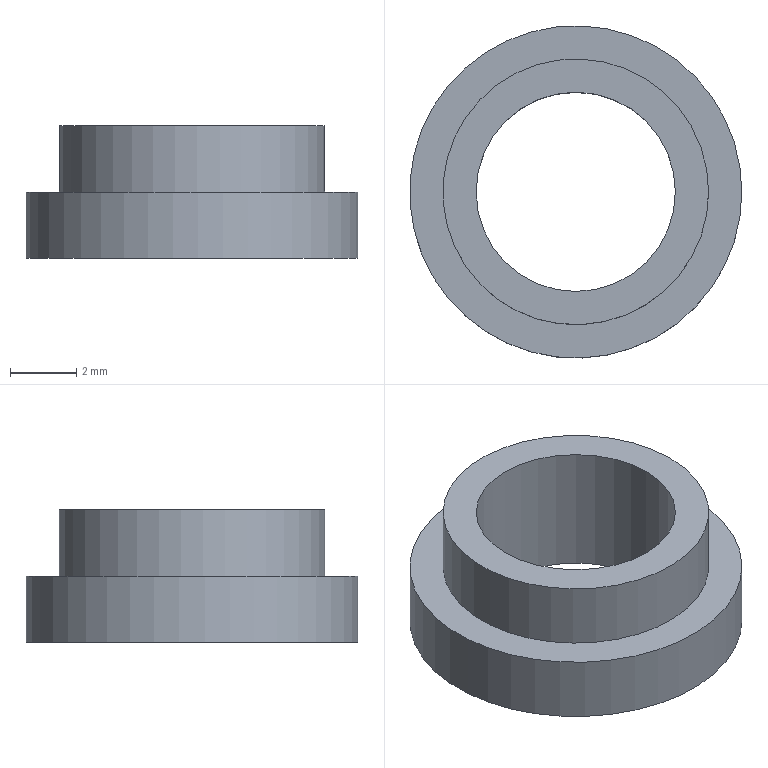Component | NX | BOTTOM_PLATE_CONNECTING_RING | 1 solid | 6 faces | box 10 x 10 x 4 mm | volume 145 mm3 | plane 3 | cylinder 3 | commonest cylinder face diameters 10 x1 8 x1 6 x1
STEP:
#1=CARTESIAN_POINT('',(0.,0.,0.));
#2=DIRECTION('',(0.,0.,1.));
#3=DIRECTION('',(1.,0.,0.));
#4=AXIS2_PLACEMENT_3D('',#1,#2,#3);
#5=CARTESIAN_POINT('',(4.,-10.,123.5));
#6=VERTEX_POINT('',#5);
#7=CARTESIAN_POINT('',(-0.,-10.,123.5));
#8=DIRECTION('',(0.,0.,1.));
#9=DIRECTION('',(1.,0.,0.));
#10=AXIS2_PLACEMENT_3D('',#7,#8,#9);
#11=CIRCLE('',#10,4.);
#12=CARTESIAN_POINT('',(-0.,-10.,123.5));
#13=DIRECTION('',(0.,0.,1.));
#14=DIRECTION('',(1.,0.,0.));
#15=AXIS2_PLACEMENT_3D('',#12,#13,#14);
#16=PLANE('',#15);
#17=CARTESIAN_POINT('',(0.,0.));
#18=DIRECTION('',(1.,0.));
#19=AXIS2_PLACEMENT_2D('',#17,#18);
#20=CIRCLE('',#19,4.);
#21=(GEOMETRIC_REPRESENTATION_CONTEXT(2)PARAMETRIC_REPRESENTATION_CONTEXT()REPRESENTATION_CONTEXT('',''));
#22=DEFINITIONAL_REPRESENTATION('',(#20),#21);
#23=PCURVE('',#16,#22);
#24=CARTESIAN_POINT('',(-0.,-10.,123.5));
#25=DIRECTION('',(0.,0.,1.));
#26=DIRECTION('',(1.,0.,0.));
#27=AXIS2_PLACEMENT_3D('',#24,#25,#26);
#28=CYLINDRICAL_SURFACE('',#27,4.);
#29=CARTESIAN_POINT('',(0.,0.));
#30=DIRECTION('',(1.,0.));
#31=VECTOR('',#30,1.);
#32=LINE('',#29,#31);
#33=(GEOMETRIC_REPRESENTATION_CONTEXT(2)PARAMETRIC_REPRESENTATION_CONTEXT()REPRESENTATION_CONTEXT('',''));
#34=DEFINITIONAL_REPRESENTATION('',(#32),#33);
#35=PCURVE('',#28,#34);
#36=SURFACE_CURVE('',#11,(#23,#35),.PCURVE_S1.);
#37=EDGE_CURVE('',#6,#6,#36,.T.);
#38=ORIENTED_EDGE('',*,*,#37,.F.);
#39=EDGE_LOOP('',(#38));
#40=FACE_BOUND('',#39,.T.);
#41=CARTESIAN_POINT('',(5.,-10.,123.5));
#42=VERTEX_POINT('',#41);
#43=CARTESIAN_POINT('',(-0.,-10.,123.5));
#44=DIRECTION('',(0.,0.,-1.));
#45=DIRECTION('',(1.,0.,0.));
#46=AXIS2_PLACEMENT_3D('',#43,#44,#45);
#47=CIRCLE('',#46,5.);
#48=CARTESIAN_POINT('',(5.,0.));
#49=CARTESIAN_POINT('',(5.,-8.66));
#50=CARTESIAN_POINT('',(-2.5,-4.33));
#51=CARTESIAN_POINT('',(-10.,-0.));
#52=CARTESIAN_POINT('',(-2.5,4.33));
#53=CARTESIAN_POINT('',(5.,8.66));
#54=CARTESIAN_POINT('',(5.,0.));
#55=(BOUNDED_CURVE()B_SPLINE_CURVE(2,(#48,#49,#50,#51,#52,#53,#54),.UNSPECIFIED.,.T.,.F.)B_SPLINE_CURVE_WITH_KNOTS((1,2,2,2,2,1),(-2.094,0.,2.094,4.189,6.283,8.378),.UNSPECIFIED.)CURVE()GEOMETRIC_REPRESENTATION_ITEM()RATIONAL_B_SPLINE_CURVE((1.,0.5,1.,0.5,1.,0.5,1.))REPRESENTATION_ITEM(''));
#56=(GEOMETRIC_REPRESENTATION_CONTEXT(2)PARAMETRIC_REPRESENTATION_CONTEXT()REPRESENTATION_CONTEXT('',''));
#57=DEFINITIONAL_REPRESENTATION('',(#55),#56);
#58=PCURVE('',#16,#57);
#59=CARTESIAN_POINT('',(-0.,-10.,121.5));
#60=DIRECTION('',(0.,0.,1.));
#61=DIRECTION('',(1.,0.,0.));
#62=AXIS2_PLACEMENT_3D('',#59,#60,#61);
#63=CYLINDRICAL_SURFACE('',#62,5.);
#64=CARTESIAN_POINT('',(6.283,2.));
#65=DIRECTION('',(-1.,0.));
#66=VECTOR('',#65,1.);
#67=LINE('',#64,#66);
#68=(GEOMETRIC_REPRESENTATION_CONTEXT(2)PARAMETRIC_REPRESENTATION_CONTEXT()REPRESENTATION_CONTEXT('',''));
#69=DEFINITIONAL_REPRESENTATION('',(#67),#68);
#70=PCURVE('',#63,#69);
#71=SURFACE_CURVE('',#47,(#58,#70),.PCURVE_S1.);
#72=EDGE_CURVE('',#42,#42,#71,.T.);
#73=ORIENTED_EDGE('',*,*,#72,.F.);
#74=EDGE_LOOP('',(#73));
#75=FACE_BOUND('',#74,.T.);
#76=ADVANCED_FACE('',(#40,#75),#16,.T.);
#77=CARTESIAN_POINT('',(3.,-10.,121.5));
#78=VERTEX_POINT('',#77);
#79=CARTESIAN_POINT('',(-0.,-10.,121.5));
#80=DIRECTION('',(0.,0.,1.));
#81=DIRECTION('',(1.,0.,0.));
#82=AXIS2_PLACEMENT_3D('',#79,#80,#81);
#83=CIRCLE('',#82,3.);
#84=CARTESIAN_POINT('',(-0.,-10.,121.5));
#85=DIRECTION('',(0.,0.,-1.));
#86=DIRECTION('',(-1.,0.,0.));
#87=AXIS2_PLACEMENT_3D('',#84,#85,#86);
#88=PLANE('',#87);
#89=CARTESIAN_POINT('',(-3.,0.));
#90=CARTESIAN_POINT('',(-3.,5.196));
#91=CARTESIAN_POINT('',(1.5,2.598));
#92=CARTESIAN_POINT('',(6.,0.));
#93=CARTESIAN_POINT('',(1.5,-2.598));
#94=CARTESIAN_POINT('',(-3.,-5.196));
#95=CARTESIAN_POINT('',(-3.,0.));
#96=(BOUNDED_CURVE()B_SPLINE_CURVE(2,(#89,#90,#91,#92,#93,#94,#95),.UNSPECIFIED.,.T.,.F.)B_SPLINE_CURVE_WITH_KNOTS((1,2,2,2,2,1),(-2.094,0.,2.094,4.189,6.283,8.378),.UNSPECIFIED.)CURVE()GEOMETRIC_REPRESENTATION_ITEM()RATIONAL_B_SPLINE_CURVE((1.,0.5,1.,0.5,1.,0.5,1.))REPRESENTATION_ITEM(''));
#97=(GEOMETRIC_REPRESENTATION_CONTEXT(2)PARAMETRIC_REPRESENTATION_CONTEXT()REPRESENTATION_CONTEXT('',''));
#98=DEFINITIONAL_REPRESENTATION('',(#96),#97);
#99=PCURVE('',#88,#98);
#100=CARTESIAN_POINT('',(-0.,-10.,126.5));
#101=DIRECTION('',(0.,0.,-1.));
#102=DIRECTION('',(-1.,0.,0.));
#103=AXIS2_PLACEMENT_3D('',#100,#101,#102);
#104=CYLINDRICAL_SURFACE('',#103,3.);
#105=CARTESIAN_POINT('',(9.425,5.));
#106=DIRECTION('',(-1.,0.));
#107=VECTOR('',#106,1.);
#108=LINE('',#105,#107);
#109=(GEOMETRIC_REPRESENTATION_CONTEXT(2)PARAMETRIC_REPRESENTATION_CONTEXT()REPRESENTATION_CONTEXT('',''));
#110=DEFINITIONAL_REPRESENTATION('',(#108),#109);
#111=PCURVE('',#104,#110);
#112=SURFACE_CURVE('',#83,(#99,#111),.PCURVE_S1.);
#113=EDGE_CURVE('',#78,#78,#112,.T.);
#114=ORIENTED_EDGE('',*,*,#113,.T.);
#115=EDGE_LOOP('',(#114));
#116=FACE_BOUND('',#115,.T.);
#117=CARTESIAN_POINT('',(5.,-10.,121.5));
#118=VERTEX_POINT('',#117);
#119=CARTESIAN_POINT('',(-0.,-10.,121.5));
#120=DIRECTION('',(0.,0.,1.));
#121=DIRECTION('',(1.,0.,0.));
#122=AXIS2_PLACEMENT_3D('',#119,#120,#121);
#123=CIRCLE('',#122,5.);
#124=CARTESIAN_POINT('',(-5.,0.));
#125=CARTESIAN_POINT('',(-5.,8.66));
#126=CARTESIAN_POINT('',(2.5,4.33));
#127=CARTESIAN_POINT('',(10.,0.));
#128=CARTESIAN_POINT('',(2.5,-4.33));
#129=CARTESIAN_POINT('',(-5.,-8.66));
#130=CARTESIAN_POINT('',(-5.,0.));
#131=(BOUNDED_CURVE()B_SPLINE_CURVE(2,(#124,#125,#126,#127,#128,#129,#130),.UNSPECIFIED.,.T.,.F.)B_SPLINE_CURVE_WITH_KNOTS((1,2,2,2,2,1),(-2.094,0.,2.094,4.189,6.283,8.378),.UNSPECIFIED.)CURVE()GEOMETRIC_REPRESENTATION_ITEM()RATIONAL_B_SPLINE_CURVE((1.,0.5,1.,0.5,1.,0.5,1.))REPRESENTATION_ITEM(''));
#132=(GEOMETRIC_REPRESENTATION_CONTEXT(2)PARAMETRIC_REPRESENTATION_CONTEXT()REPRESENTATION_CONTEXT('',''));
#133=DEFINITIONAL_REPRESENTATION('',(#131),#132);
#134=PCURVE('',#88,#133);
#135=CARTESIAN_POINT('',(0.,0.));
#136=DIRECTION('',(1.,0.));
#137=VECTOR('',#136,1.);
#138=LINE('',#135,#137);
#139=(GEOMETRIC_REPRESENTATION_CONTEXT(2)PARAMETRIC_REPRESENTATION_CONTEXT()REPRESENTATION_CONTEXT('',''));
#140=DEFINITIONAL_REPRESENTATION('',(#138),#139);
#141=PCURVE('',#63,#140);
#142=SURFACE_CURVE('',#123,(#134,#141),.PCURVE_S1.);
#143=EDGE_CURVE('',#118,#118,#142,.T.);
#144=ORIENTED_EDGE('',*,*,#143,.F.);
#145=EDGE_LOOP('',(#144));
#146=FACE_BOUND('',#145,.T.);
#147=ADVANCED_FACE('',(#116,#146),#88,.T.);
#148=ORIENTED_EDGE('',*,*,#72,.T.);
#149=CARTESIAN_POINT('',(5.,-10.,121.5));
#150=CARTESIAN_POINT('',(5.,-10.,123.5));
#151=B_SPLINE_CURVE_WITH_KNOTS('',1,(#149,#150),.UNSPECIFIED.,.F.,.F.,(2,2),(0.,2.),.PIECEWISE_BEZIER_KNOTS.);
#152=CARTESIAN_POINT('',(0.,0.));
#153=DIRECTION('',(0.,1.));
#154=VECTOR('',#153,1.);
#155=LINE('',#152,#154);
#156=(GEOMETRIC_REPRESENTATION_CONTEXT(2)PARAMETRIC_REPRESENTATION_CONTEXT()REPRESENTATION_CONTEXT('',''));
#157=DEFINITIONAL_REPRESENTATION('',(#155),#156);
#158=PCURVE('',#63,#157);
#159=CARTESIAN_POINT('',(6.283,0.));
#160=DIRECTION('',(0.,1.));
#161=VECTOR('',#160,1.);
#162=LINE('',#159,#161);
#163=(GEOMETRIC_REPRESENTATION_CONTEXT(2)PARAMETRIC_REPRESENTATION_CONTEXT()REPRESENTATION_CONTEXT('',''));
#164=DEFINITIONAL_REPRESENTATION('',(#162),#163);
#165=PCURVE('',#63,#164);
#166=SEAM_CURVE('',#151,(#158,#165),.PCURVE_S1.);
#167=EDGE_CURVE('',#118,#42,#166,.T.);
#168=ORIENTED_EDGE('',*,*,#167,.F.);
#169=ORIENTED_EDGE('',*,*,#143,.T.);
#170=ORIENTED_EDGE('',*,*,#167,.T.);
#171=EDGE_LOOP('',(#148,#168,#169,#170));
#172=FACE_BOUND('',#171,.T.);
#173=ADVANCED_FACE('',(#172),#63,.T.);
#174=CARTESIAN_POINT('',(3.,-10.,125.5));
#175=VERTEX_POINT('',#174);
#176=CARTESIAN_POINT('',(-0.,-10.,125.5));
#177=DIRECTION('',(0.,0.,-1.));
#178=DIRECTION('',(1.,0.,0.));
#179=AXIS2_PLACEMENT_3D('',#176,#177,#178);
#180=CIRCLE('',#179,3.);
#181=CARTESIAN_POINT('',(-0.,-10.,125.5));
#182=DIRECTION('',(0.,0.,1.));
#183=DIRECTION('',(1.,0.,0.));
#184=AXIS2_PLACEMENT_3D('',#181,#182,#183);
#185=PLANE('',#184);
#186=CARTESIAN_POINT('',(3.,0.));
#187=CARTESIAN_POINT('',(3.,-5.196));
#188=CARTESIAN_POINT('',(-1.5,-2.598));
#189=CARTESIAN_POINT('',(-6.,-0.));
#190=CARTESIAN_POINT('',(-1.5,2.598));
#191=CARTESIAN_POINT('',(3.,5.196));
#192=CARTESIAN_POINT('',(3.,0.));
#193=(BOUNDED_CURVE()B_SPLINE_CURVE(2,(#186,#187,#188,#189,#190,#191,#192),.UNSPECIFIED.,.T.,.F.)B_SPLINE_CURVE_WITH_KNOTS((1,2,2,2,2,1),(-2.094,0.,2.094,4.189,6.283,8.378),.UNSPECIFIED.)CURVE()GEOMETRIC_REPRESENTATION_ITEM()RATIONAL_B_SPLINE_CURVE((1.,0.5,1.,0.5,1.,0.5,1.))REPRESENTATION_ITEM(''));
#194=(GEOMETRIC_REPRESENTATION_CONTEXT(2)PARAMETRIC_REPRESENTATION_CONTEXT()REPRESENTATION_CONTEXT('',''));
#195=DEFINITIONAL_REPRESENTATION('',(#193),#194);
#196=PCURVE('',#185,#195);
#197=CARTESIAN_POINT('',(3.142,1.));
#198=DIRECTION('',(1.,0.));
#199=VECTOR('',#198,1.);
#200=LINE('',#197,#199);
#201=(GEOMETRIC_REPRESENTATION_CONTEXT(2)PARAMETRIC_REPRESENTATION_CONTEXT()REPRESENTATION_CONTEXT('',''));
#202=DEFINITIONAL_REPRESENTATION('',(#200),#201);
#203=PCURVE('',#104,#202);
#204=SURFACE_CURVE('',#180,(#196,#203),.PCURVE_S1.);
#205=EDGE_CURVE('',#175,#175,#204,.T.);
#206=ORIENTED_EDGE('',*,*,#205,.T.);
#207=EDGE_LOOP('',(#206));
#208=FACE_BOUND('',#207,.T.);
#209=CARTESIAN_POINT('',(4.,-10.,125.5));
#210=VERTEX_POINT('',#209);
#211=CARTESIAN_POINT('',(-0.,-10.,125.5));
#212=DIRECTION('',(0.,0.,1.));
#213=DIRECTION('',(1.,0.,0.));
#214=AXIS2_PLACEMENT_3D('',#211,#212,#213);
#215=CIRCLE('',#214,4.);
#216=CARTESIAN_POINT('',(0.,0.));
#217=DIRECTION('',(1.,0.));
#218=AXIS2_PLACEMENT_2D('',#216,#217);
#219=CIRCLE('',#218,4.);
#220=(GEOMETRIC_REPRESENTATION_CONTEXT(2)PARAMETRIC_REPRESENTATION_CONTEXT()REPRESENTATION_CONTEXT('',''));
#221=DEFINITIONAL_REPRESENTATION('',(#219),#220);
#222=PCURVE('',#185,#221);
#223=CARTESIAN_POINT('',(0.,2.));
#224=DIRECTION('',(1.,0.));
#225=VECTOR('',#224,1.);
#226=LINE('',#223,#225);
#227=(GEOMETRIC_REPRESENTATION_CONTEXT(2)PARAMETRIC_REPRESENTATION_CONTEXT()REPRESENTATION_CONTEXT('',''));
#228=DEFINITIONAL_REPRESENTATION('',(#226),#227);
#229=PCURVE('',#28,#228);
#230=SURFACE_CURVE('',#215,(#222,#229),.PCURVE_S1.);
#231=EDGE_CURVE('',#210,#210,#230,.T.);
#232=ORIENTED_EDGE('',*,*,#231,.T.);
#233=EDGE_LOOP('',(#232));
#234=FACE_BOUND('',#233,.T.);
#235=ADVANCED_FACE('',(#208,#234),#185,.T.);
#236=ORIENTED_EDGE('',*,*,#231,.F.);
#237=CARTESIAN_POINT('',(4.,-10.,123.5));
#238=CARTESIAN_POINT('',(4.,-10.,125.5));
#239=B_SPLINE_CURVE_WITH_KNOTS('',1,(#237,#238),.UNSPECIFIED.,.F.,.F.,(2,2),(0.,2.),.PIECEWISE_BEZIER_KNOTS.);
#240=CARTESIAN_POINT('',(0.,0.));
#241=DIRECTION('',(0.,1.));
#242=VECTOR('',#241,1.);
#243=LINE('',#240,#242);
#244=(GEOMETRIC_REPRESENTATION_CONTEXT(2)PARAMETRIC_REPRESENTATION_CONTEXT()REPRESENTATION_CONTEXT('',''));
#245=DEFINITIONAL_REPRESENTATION('',(#243),#244);
#246=PCURVE('',#28,#245);
#247=CARTESIAN_POINT('',(6.283,0.));
#248=DIRECTION('',(0.,1.));
#249=VECTOR('',#248,1.);
#250=LINE('',#247,#249);
#251=(GEOMETRIC_REPRESENTATION_CONTEXT(2)PARAMETRIC_REPRESENTATION_CONTEXT()REPRESENTATION_CONTEXT('',''));
#252=DEFINITIONAL_REPRESENTATION('',(#250),#251);
#253=PCURVE('',#28,#252);
#254=SEAM_CURVE('',#239,(#246,#253),.PCURVE_S1.);
#255=EDGE_CURVE('',#6,#210,#254,.T.);
#256=ORIENTED_EDGE('',*,*,#255,.F.);
#257=ORIENTED_EDGE('',*,*,#37,.T.);
#258=ORIENTED_EDGE('',*,*,#255,.T.);
#259=EDGE_LOOP('',(#236,#256,#257,#258));
#260=FACE_BOUND('',#259,.T.);
#261=ADVANCED_FACE('',(#260),#28,.T.);
#262=ORIENTED_EDGE('',*,*,#205,.T.);
#263=CARTESIAN_POINT('',(3.,-10.,125.5));
#264=CARTESIAN_POINT('',(3.,-10.,121.5));
#265=B_SPLINE_CURVE_WITH_KNOTS('',1,(#263,#264),.UNSPECIFIED.,.F.,.F.,(2,2),(1.,5.),.PIECEWISE_BEZIER_KNOTS.);
#266=CARTESIAN_POINT('',(9.425,0.));
#267=DIRECTION('',(0.,1.));
#268=VECTOR('',#267,1.);
#269=LINE('',#266,#268);
#270=(GEOMETRIC_REPRESENTATION_CONTEXT(2)PARAMETRIC_REPRESENTATION_CONTEXT()REPRESENTATION_CONTEXT('',''));
#271=DEFINITIONAL_REPRESENTATION('',(#269),#270);
#272=PCURVE('',#104,#271);
#273=CARTESIAN_POINT('',(3.142,0.));
#274=DIRECTION('',(0.,1.));
#275=VECTOR('',#274,1.);
#276=LINE('',#273,#275);
#277=(GEOMETRIC_REPRESENTATION_CONTEXT(2)PARAMETRIC_REPRESENTATION_CONTEXT()REPRESENTATION_CONTEXT('',''));
#278=DEFINITIONAL_REPRESENTATION('',(#276),#277);
#279=PCURVE('',#104,#278);
#280=SEAM_CURVE('',#265,(#272,#279),.PCURVE_S1.);
#281=EDGE_CURVE('',#175,#78,#280,.T.);
#282=ORIENTED_EDGE('',*,*,#281,.T.);
#283=ORIENTED_EDGE('',*,*,#113,.T.);
#284=ORIENTED_EDGE('',*,*,#281,.F.);
#285=EDGE_LOOP('',(#262,#282,#283,#284));
#286=FACE_BOUND('',#285,.F.);
#287=ADVANCED_FACE('',(#286),#104,.F.);
#288=CLOSED_SHELL('',(#76,#147,#173,#235,#261,#287));
#289=MANIFOLD_SOLID_BREP('',#288);
#290=(LENGTH_UNIT()NAMED_UNIT(*)SI_UNIT(.MILLI.,.METRE.));
#291=UNCERTAINTY_MEASURE_WITH_UNIT(LENGTH_MEASURE(0.00001),#290,'','');
#292=(NAMED_UNIT(*)PLANE_ANGLE_UNIT()SI_UNIT($,.RADIAN.));
#293=(NAMED_UNIT(*)SI_UNIT($,.STERADIAN.)SOLID_ANGLE_UNIT());
#294=(GEOMETRIC_REPRESENTATION_CONTEXT(3)GLOBAL_UNCERTAINTY_ASSIGNED_CONTEXT((#291))GLOBAL_UNIT_ASSIGNED_CONTEXT((#290,#292,#293))REPRESENTATION_CONTEXT('',''));
#295=ADVANCED_BREP_SHAPE_REPRESENTATION('',(#4,#289),#294);